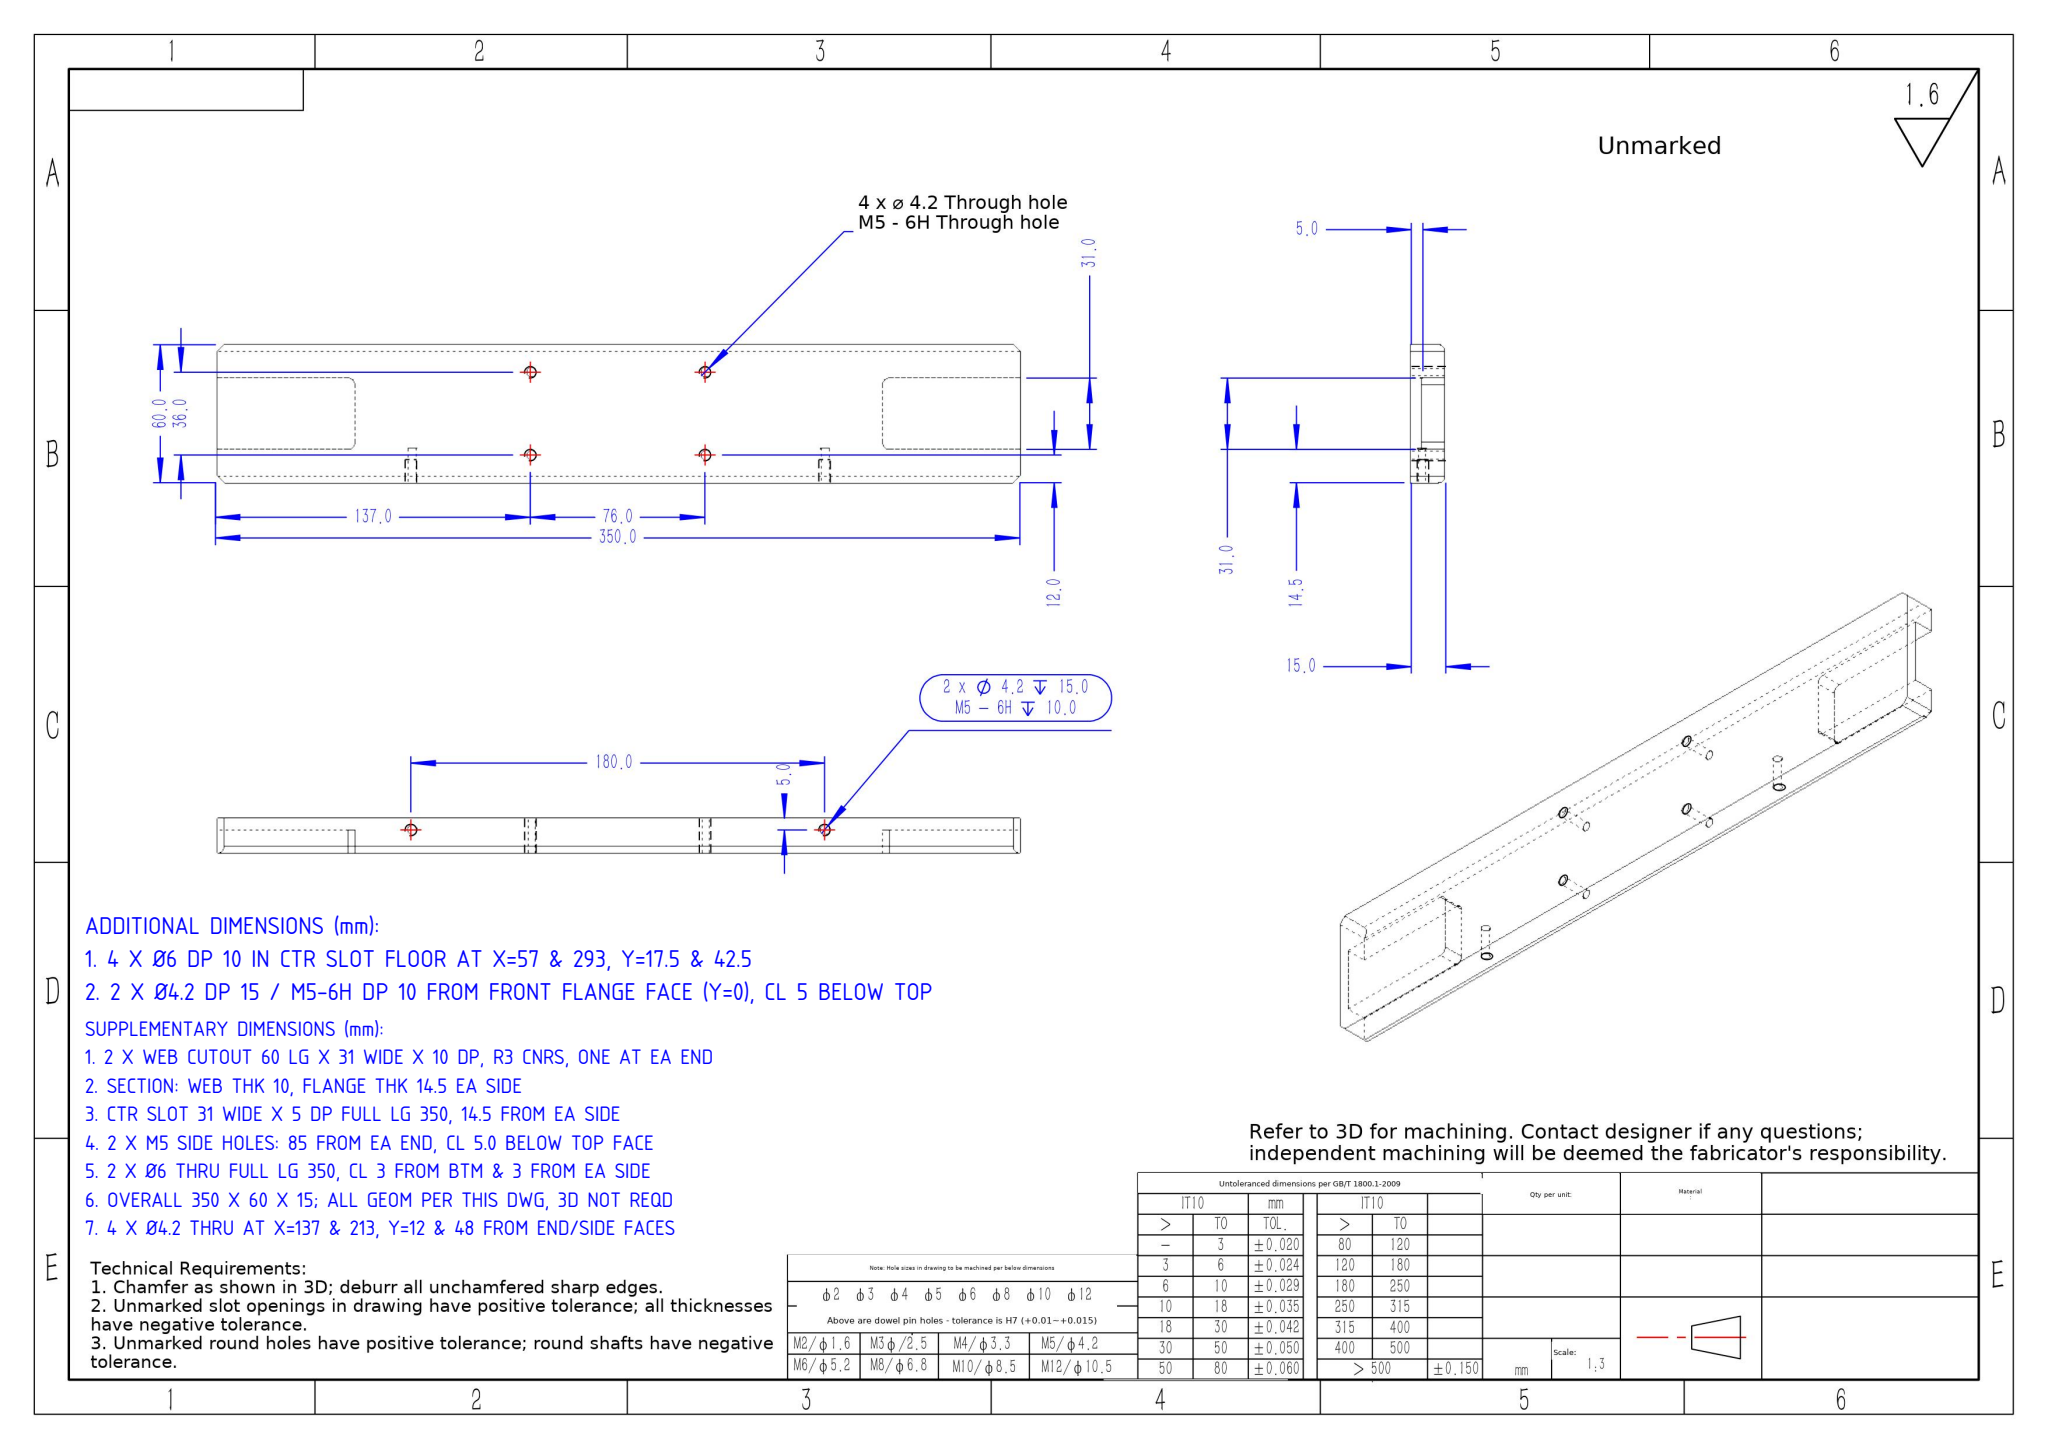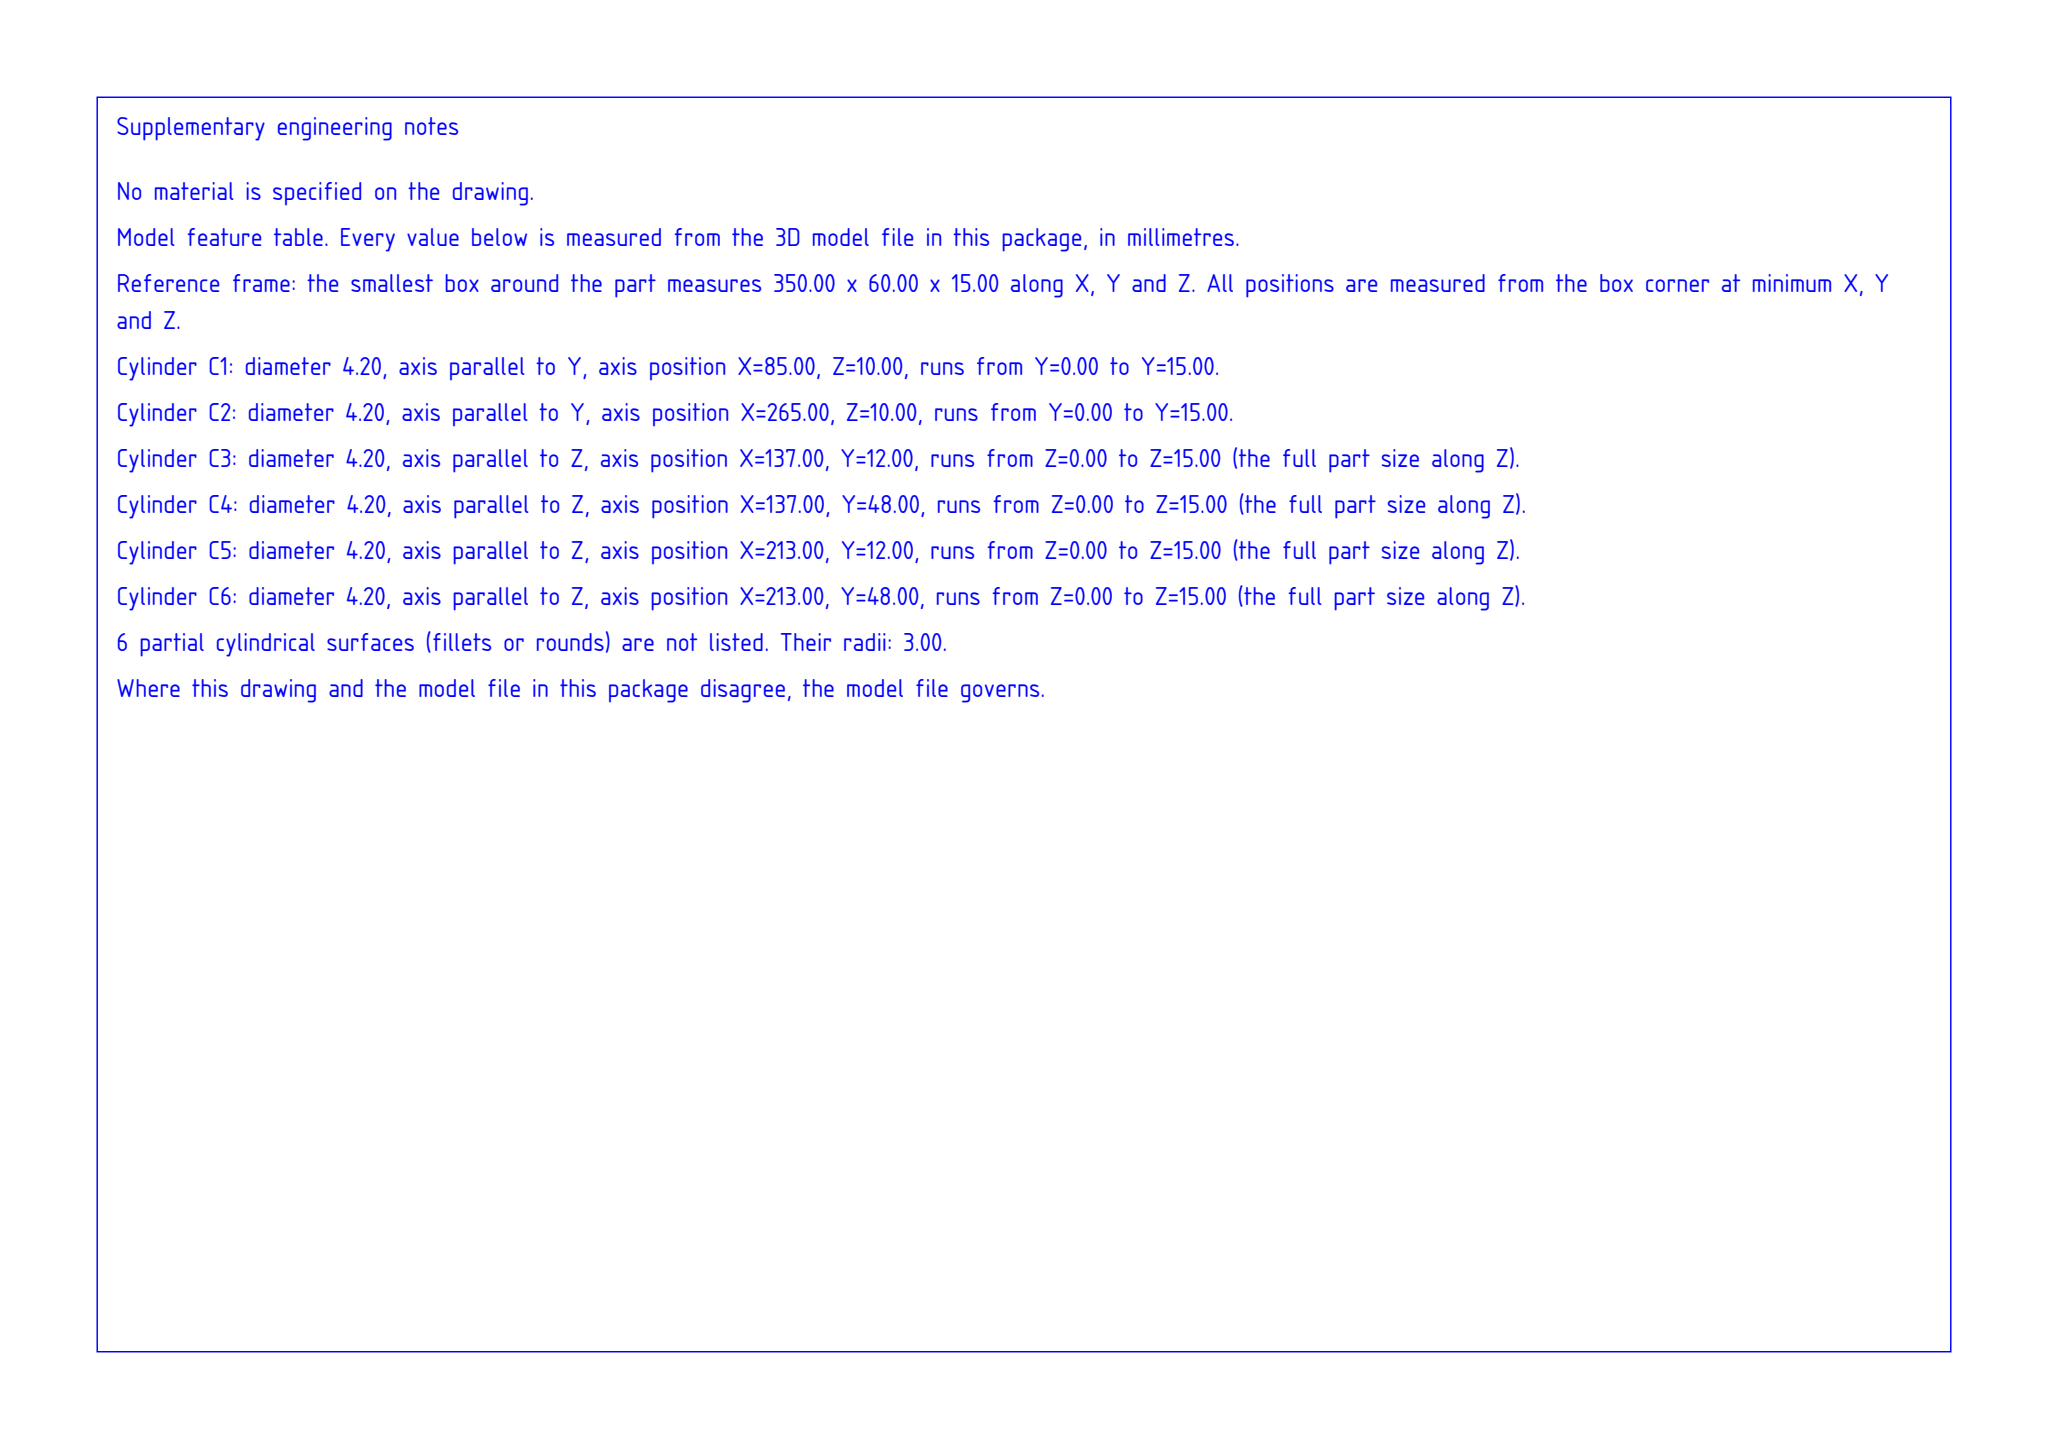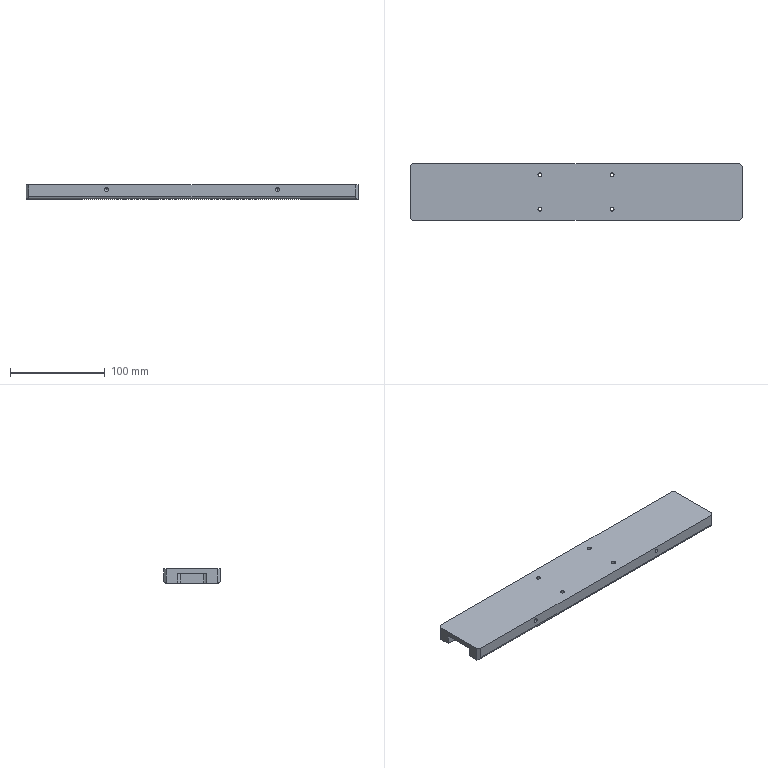Part | SolidWorks | mm | 1 solid | 40 faces | box 350 x 60 x 15 mm | volume 275015 mm3 | cylinder 18 | plane 18 | cone 4 | commonest cylinder face diameters 4.2 x12 6 x6
build123d program:
from build123d import *

# Parameters (mm, degrees)
SKETCH1_W             = 350
SKETCH1_H             = 60
BOSS_EXTRUDE1_DEPTH   = 7.5
M5_TAPPED_HOLE1_D     = 4.2
CHAMFER1_SIZE         = 3
SKETCH4_W             = 60
SKETCH4_H             = 31
CUT_EXTRUDE1_DEPTH    = 10
FILLET1_R             = 3
FILLET1_OF_MIRROR1_R  = 3
FILLET2_R             = 3
M5_TAPPED_HOLE2_D     = 4.2
M5_TAPPED_HOLE2_DEPTH = 15
M5_TAPPED_HOLE2_TIP   = 1.262


with BuildPart() as part:
    # Sketch1 → Boss-Extrude1 (new, symmetric)
    with BuildSketch(Plane.XY):
        Rectangle(SKETCH1_W, SKETCH1_H)
    extrude(amount=BOSS_EXTRUDE1_DEPTH, both=True)

    # M5 Tapped Hole1 (through all)
    with Locations(Plane.XY.offset(7.5)):
        with Locations((-38, 18), (-38, -18), (38, -18), (38, 18)):
            Hole(M5_TAPPED_HOLE1_D / 2)

    # Chamfer1
    chamfer1_edges = [part.edges().sort_by_distance(p)[0] for p in [
        (175, -30, 0),
        (-175, -30, 0),
        (-175, 30, 0),
        (175, 30, 0),
    ]]
    chamfer(chamfer1_edges, length=CHAMFER1_SIZE)

    # Sketch4 → Cut-Extrude1 (cut)
    with BuildSketch(Plane(origin=(0, 0, -7.5), x_dir=(-1, 0, 0), z_dir=(0, 0, -1))):
        with Locations((-145, 0)):
            Rectangle(SKETCH4_W, SKETCH4_H)
    cut_extrude1 = extrude(amount=-CUT_EXTRUDE1_DEPTH, mode=Mode.SUBTRACT)

    # Fillet1
    fillet1_edges = [part.edges().sort_by_distance(p)[0] for p in [
        (115, 15.5, -2.5),
        (115, -15.5, -2.5),
    ]]
    fillet(fillet1_edges, radius=FILLET1_R)

    # Mirror1: Cut-Extrude1 across plane
    add(cut_extrude1.mirror(Plane(origin=(0, 0, 0), x_dir=(0, 0, 1), z_dir=(1, 0, 0))), mode=Mode.SUBTRACT)

    # Fillet1 of Mirror1
    fillet1_of_mirror1_edges = [part.edges().sort_by_distance(p)[0] for p in [
        (-115, 15.5, -2.5),
        (-115, -15.5, -2.5),
    ]]
    fillet(fillet1_of_mirror1_edges, radius=FILLET1_OF_MIRROR1_R)

    # Fillet2
    fillet2_edges = [part.edges().sort_by_distance(p)[0] for p in [
        (0, 30, -7.5),
        (0, -30, -7.5),
    ]]
    fillet(fillet2_edges, radius=FILLET2_R)

    # M5 Tapped Hole2
    with Locations(Plane(origin=(0, -30, 0), x_dir=(-1, 0, 0), z_dir=(0, -1, 0))):
        with Locations((90, -2.5), (-90, -2.5)):
            Hole(M5_TAPPED_HOLE2_D / 2, depth=M5_TAPPED_HOLE2_DEPTH)
            with Locations((0, 0, -(M5_TAPPED_HOLE2_DEPTH + M5_TAPPED_HOLE2_TIP / 2))):  # 118° drill point
                Cone(0, M5_TAPPED_HOLE2_D / 2, M5_TAPPED_HOLE2_TIP, mode=Mode.SUBTRACT)


solid = part.part